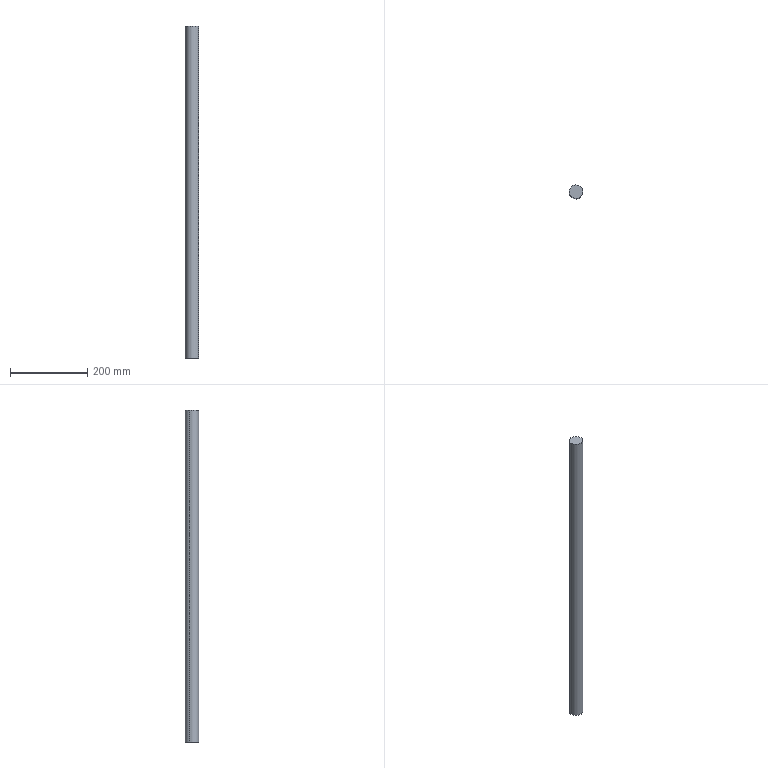Component | SolidWorks | PistonRod-1 | 1 solid | 4 faces | box 35 x 35 x 860 mm | volume 827417 mm3 | cylinder 2 | plane 2 | commonest cylinder face diameters 35 x2
build123d program:
from build123d import *

# Parameters (mm, degrees)
SKETCH1_R           = 17.5
BOSS_EXTRUDE1_DEPTH = 430


with BuildPart() as part:
    # Sketch1 → Boss-Extrude1 (new, symmetric)
    with BuildSketch(Plane.XY):
        Circle(SKETCH1_R)
    extrude(amount=BOSS_EXTRUDE1_DEPTH, both=True)


solid = part.part

# Placed as in the assembly
solid = solid.moved(Location((-7.456, 2.584, 805), (0, 0, 0)))
STEP:
#1=COLOUR_RGB('',0.7922,0.8196,0.9333);
#2=FILL_AREA_STYLE_COLOUR('',#1);
#3=FILL_AREA_STYLE('',(#2));
#4=SURFACE_STYLE_FILL_AREA(#3);
#5=SURFACE_SIDE_STYLE('',(#4));
#6=SURFACE_STYLE_USAGE(.BOTH.,#5);
#7=PRESENTATION_STYLE_ASSIGNMENT((#6));
#8=CARTESIAN_POINT('',(-0.9493,0.313,48.622));
#9=VERTEX_POINT('',#8);
#10=CARTESIAN_POINT('',(0.3622,-0.1096,48.622));
#11=VERTEX_POINT('',#10);
#12=CARTESIAN_POINT('',(-0.2935,0.1017,48.622));
#13=DIRECTION('',(0.,0.,1.));
#14=DIRECTION('',(-0.9518,0.3067,0.));
#15=AXIS2_PLACEMENT_3D('',#12,#13,#14);
#16=CIRCLE('',#15,0.689);
#17=EDGE_CURVE('',#9,#11,#16,.T.);
#18=ORIENTED_EDGE('',*,*,#17,.F.);
#19=CARTESIAN_POINT('',(-0.9493,0.313,14.764));
#20=VERTEX_POINT('',#19);
#21=CARTESIAN_POINT('',(-0.9493,0.313,48.622));
#22=DIRECTION('',(0.,0.,-1.));
#23=VECTOR('',#22,39.37);
#24=LINE('',#21,#23);
#25=EDGE_CURVE('',#9,#20,#24,.T.);
#26=ORIENTED_EDGE('',*,*,#25,.T.);
#27=CARTESIAN_POINT('',(0.3622,-0.1096,14.764));
#28=VERTEX_POINT('',#27);
#29=CARTESIAN_POINT('',(-0.2935,0.1017,14.764));
#30=DIRECTION('',(0.,0.,1.));
#31=DIRECTION('',(-0.9518,0.3067,0.));
#32=AXIS2_PLACEMENT_3D('',#29,#30,#31);
#33=CIRCLE('',#32,0.689);
#34=EDGE_CURVE('',#20,#28,#33,.T.);
#35=ORIENTED_EDGE('',*,*,#34,.T.);
#36=CARTESIAN_POINT('',(0.3622,-0.1096,48.622));
#37=DIRECTION('',(0.,0.,-1.));
#38=VECTOR('',#37,39.37);
#39=LINE('',#36,#38);
#40=EDGE_CURVE('',#11,#28,#39,.T.);
#41=ORIENTED_EDGE('',*,*,#40,.F.);
#42=EDGE_LOOP('',(#18,#26,#35,#41));
#43=FACE_OUTER_BOUND('',#42,.T.);
#44=CARTESIAN_POINT('',(-0.2935,0.1017,48.622));
#45=DIRECTION('',(0.,0.,-1.));
#46=DIRECTION('',(0.9518,-0.3067,0.));
#47=AXIS2_PLACEMENT_3D('',#44,#45,#46);
#48=CYLINDRICAL_SURFACE('',#47,0.689);
#49=ADVANCED_FACE('',(#43),#48,.T.);
#50=ORIENTED_EDGE('',*,*,#25,.F.);
#51=CARTESIAN_POINT('',(-0.2935,0.1017,48.622));
#52=DIRECTION('',(0.,0.,1.));
#53=DIRECTION('',(-0.9518,0.3067,0.));
#54=AXIS2_PLACEMENT_3D('',#51,#52,#53);
#55=CIRCLE('',#54,0.689);
#56=EDGE_CURVE('',#11,#9,#55,.T.);
#57=ORIENTED_EDGE('',*,*,#56,.F.);
#58=ORIENTED_EDGE('',*,*,#40,.T.);
#59=CARTESIAN_POINT('',(-0.2935,0.1017,14.764));
#60=DIRECTION('',(0.,0.,1.));
#61=DIRECTION('',(-0.9518,0.3067,0.));
#62=AXIS2_PLACEMENT_3D('',#59,#60,#61);
#63=CIRCLE('',#62,0.689);
#64=EDGE_CURVE('',#28,#20,#63,.T.);
#65=ORIENTED_EDGE('',*,*,#64,.T.);
#66=EDGE_LOOP('',(#50,#57,#58,#65));
#67=FACE_OUTER_BOUND('',#66,.T.);
#68=CARTESIAN_POINT('',(-0.2935,0.1017,48.622));
#69=DIRECTION('',(0.,0.,-1.));
#70=DIRECTION('',(0.9518,-0.3067,0.));
#71=AXIS2_PLACEMENT_3D('',#68,#69,#70);
#72=CYLINDRICAL_SURFACE('',#71,0.689);
#73=ADVANCED_FACE('',(#67),#72,.T.);
#74=ORIENTED_EDGE('',*,*,#56,.T.);
#75=ORIENTED_EDGE('',*,*,#17,.T.);
#76=EDGE_LOOP('',(#74,#75));
#77=FACE_OUTER_BOUND('',#76,.T.);
#78=CARTESIAN_POINT('',(-0.2935,0.1017,48.622));
#79=DIRECTION('',(0.,0.,1.));
#80=DIRECTION('',(-0.9518,0.3067,0.));
#81=AXIS2_PLACEMENT_3D('',#78,#79,#80);
#82=PLANE('',#81);
#83=ADVANCED_FACE('',(#77),#82,.T.);
#84=ORIENTED_EDGE('',*,*,#64,.F.);
#85=ORIENTED_EDGE('',*,*,#34,.F.);
#86=EDGE_LOOP('',(#84,#85));
#87=FACE_OUTER_BOUND('',#86,.T.);
#88=CARTESIAN_POINT('',(-0.2935,0.1017,14.764));
#89=DIRECTION('',(0.,0.,1.));
#90=DIRECTION('',(-0.9518,0.3067,0.));
#91=AXIS2_PLACEMENT_3D('',#88,#89,#90);
#92=PLANE('',#91);
#93=ADVANCED_FACE('',(#87),#92,.F.);
#94=CLOSED_SHELL('',(#49,#73,#83,#93));
#95=MANIFOLD_SOLID_BREP('',#94);
#96=STYLED_ITEM('',(#7),#95);
#97=PRESENTATION_LAYER_ASSIGNMENT('','',(#96));
#98=(LENGTH_UNIT()NAMED_UNIT(*)SI_UNIT($,.METRE.));
#99=LENGTH_MEASURE_WITH_UNIT(LENGTH_MEASURE(0.0254),#98);
#100=DIMENSIONAL_EXPONENTS(1.,0.,0.,0.,0.,0.,0.);
#101=(CONVERSION_BASED_UNIT('',#99)LENGTH_UNIT()NAMED_UNIT(#100));
#102=UNCERTAINTY_MEASURE_WITH_UNIT(LENGTH_MEASURE(0.00001),#101,'','');
#103=(NAMED_UNIT(*)PLANE_ANGLE_UNIT()SI_UNIT($,.RADIAN.));
#104=(NAMED_UNIT(*)SI_UNIT($,.STERADIAN.)SOLID_ANGLE_UNIT());
#105=(GEOMETRIC_REPRESENTATION_CONTEXT(3)GLOBAL_UNCERTAINTY_ASSIGNED_CONTEXT((#102))GLOBAL_UNIT_ASSIGNED_CONTEXT((#101,#103,#104))REPRESENTATION_CONTEXT('',''));
#106=MECHANICAL_DESIGN_GEOMETRIC_PRESENTATION_REPRESENTATION('',(#96),#105);
#107=CARTESIAN_POINT('',(0.,0.,0.));
#108=DIRECTION('',(0.,0.,1.));
#109=DIRECTION('',(1.,0.,0.));
#110=AXIS2_PLACEMENT_3D('',#107,#108,#109);
#111=(LENGTH_UNIT()NAMED_UNIT(*)SI_UNIT($,.METRE.));
#112=LENGTH_MEASURE_WITH_UNIT(LENGTH_MEASURE(0.0254),#111);
#113=DIMENSIONAL_EXPONENTS(1.,0.,0.,0.,0.,0.,0.);
#114=(CONVERSION_BASED_UNIT('',#112)LENGTH_UNIT()NAMED_UNIT(#113));
#115=UNCERTAINTY_MEASURE_WITH_UNIT(LENGTH_MEASURE(0.00001),#114,'','');
#116=(NAMED_UNIT(*)PLANE_ANGLE_UNIT()SI_UNIT($,.RADIAN.));
#117=(NAMED_UNIT(*)SI_UNIT($,.STERADIAN.)SOLID_ANGLE_UNIT());
#118=(GEOMETRIC_REPRESENTATION_CONTEXT(3)GLOBAL_UNCERTAINTY_ASSIGNED_CONTEXT((#115))GLOBAL_UNIT_ASSIGNED_CONTEXT((#114,#116,#117))REPRESENTATION_CONTEXT('',''));
#119=ADVANCED_BREP_SHAPE_REPRESENTATION('',(#95,#110),#118);